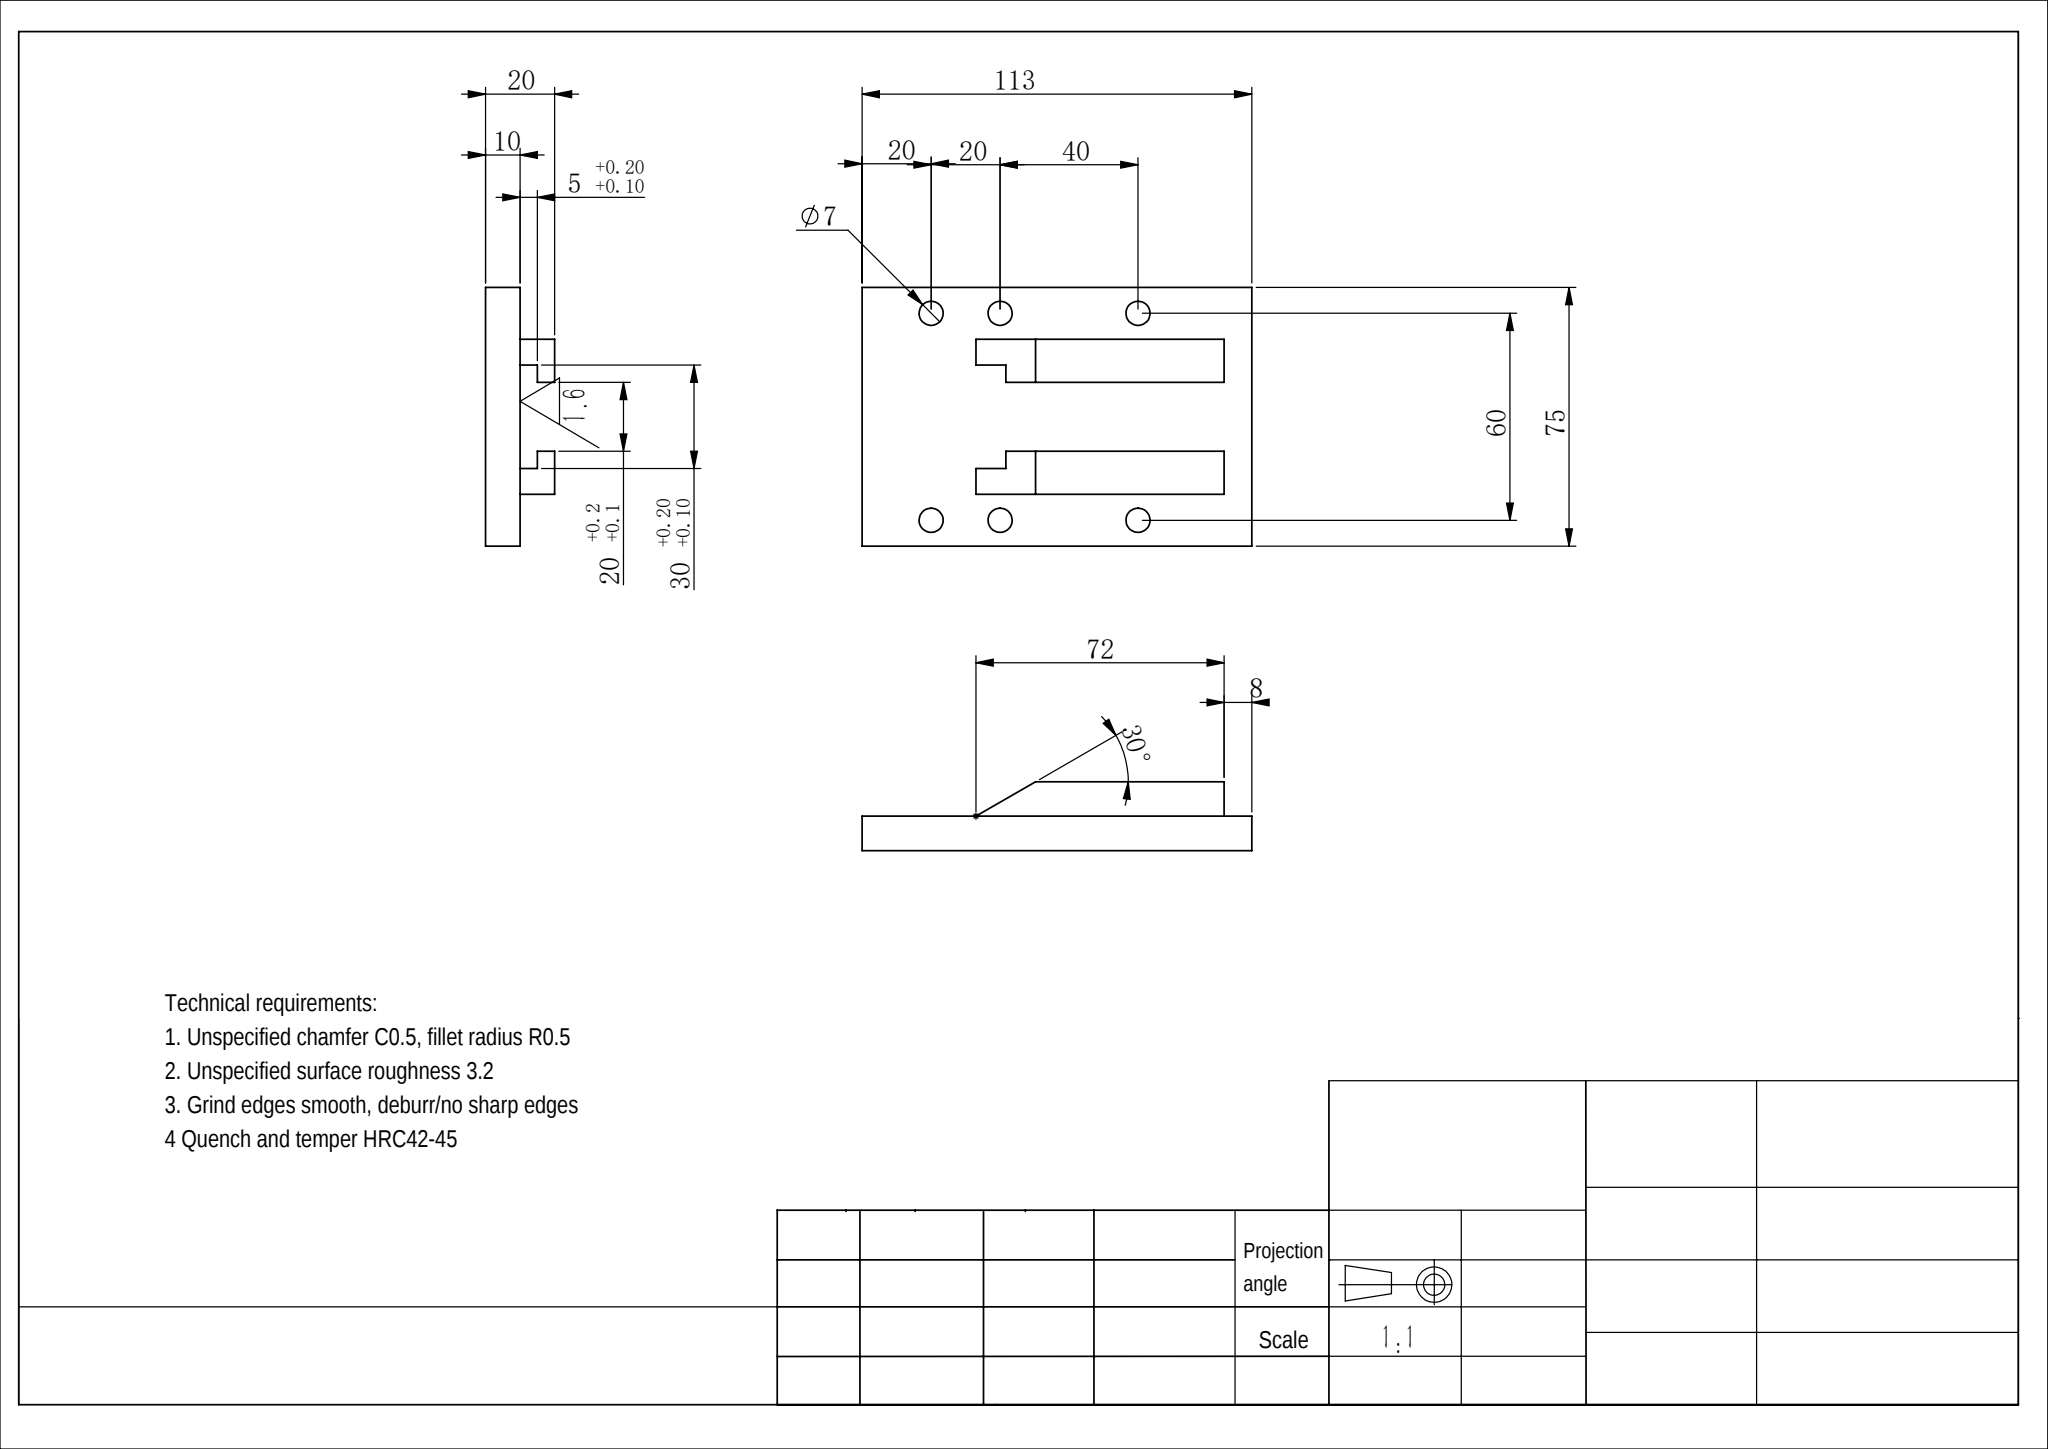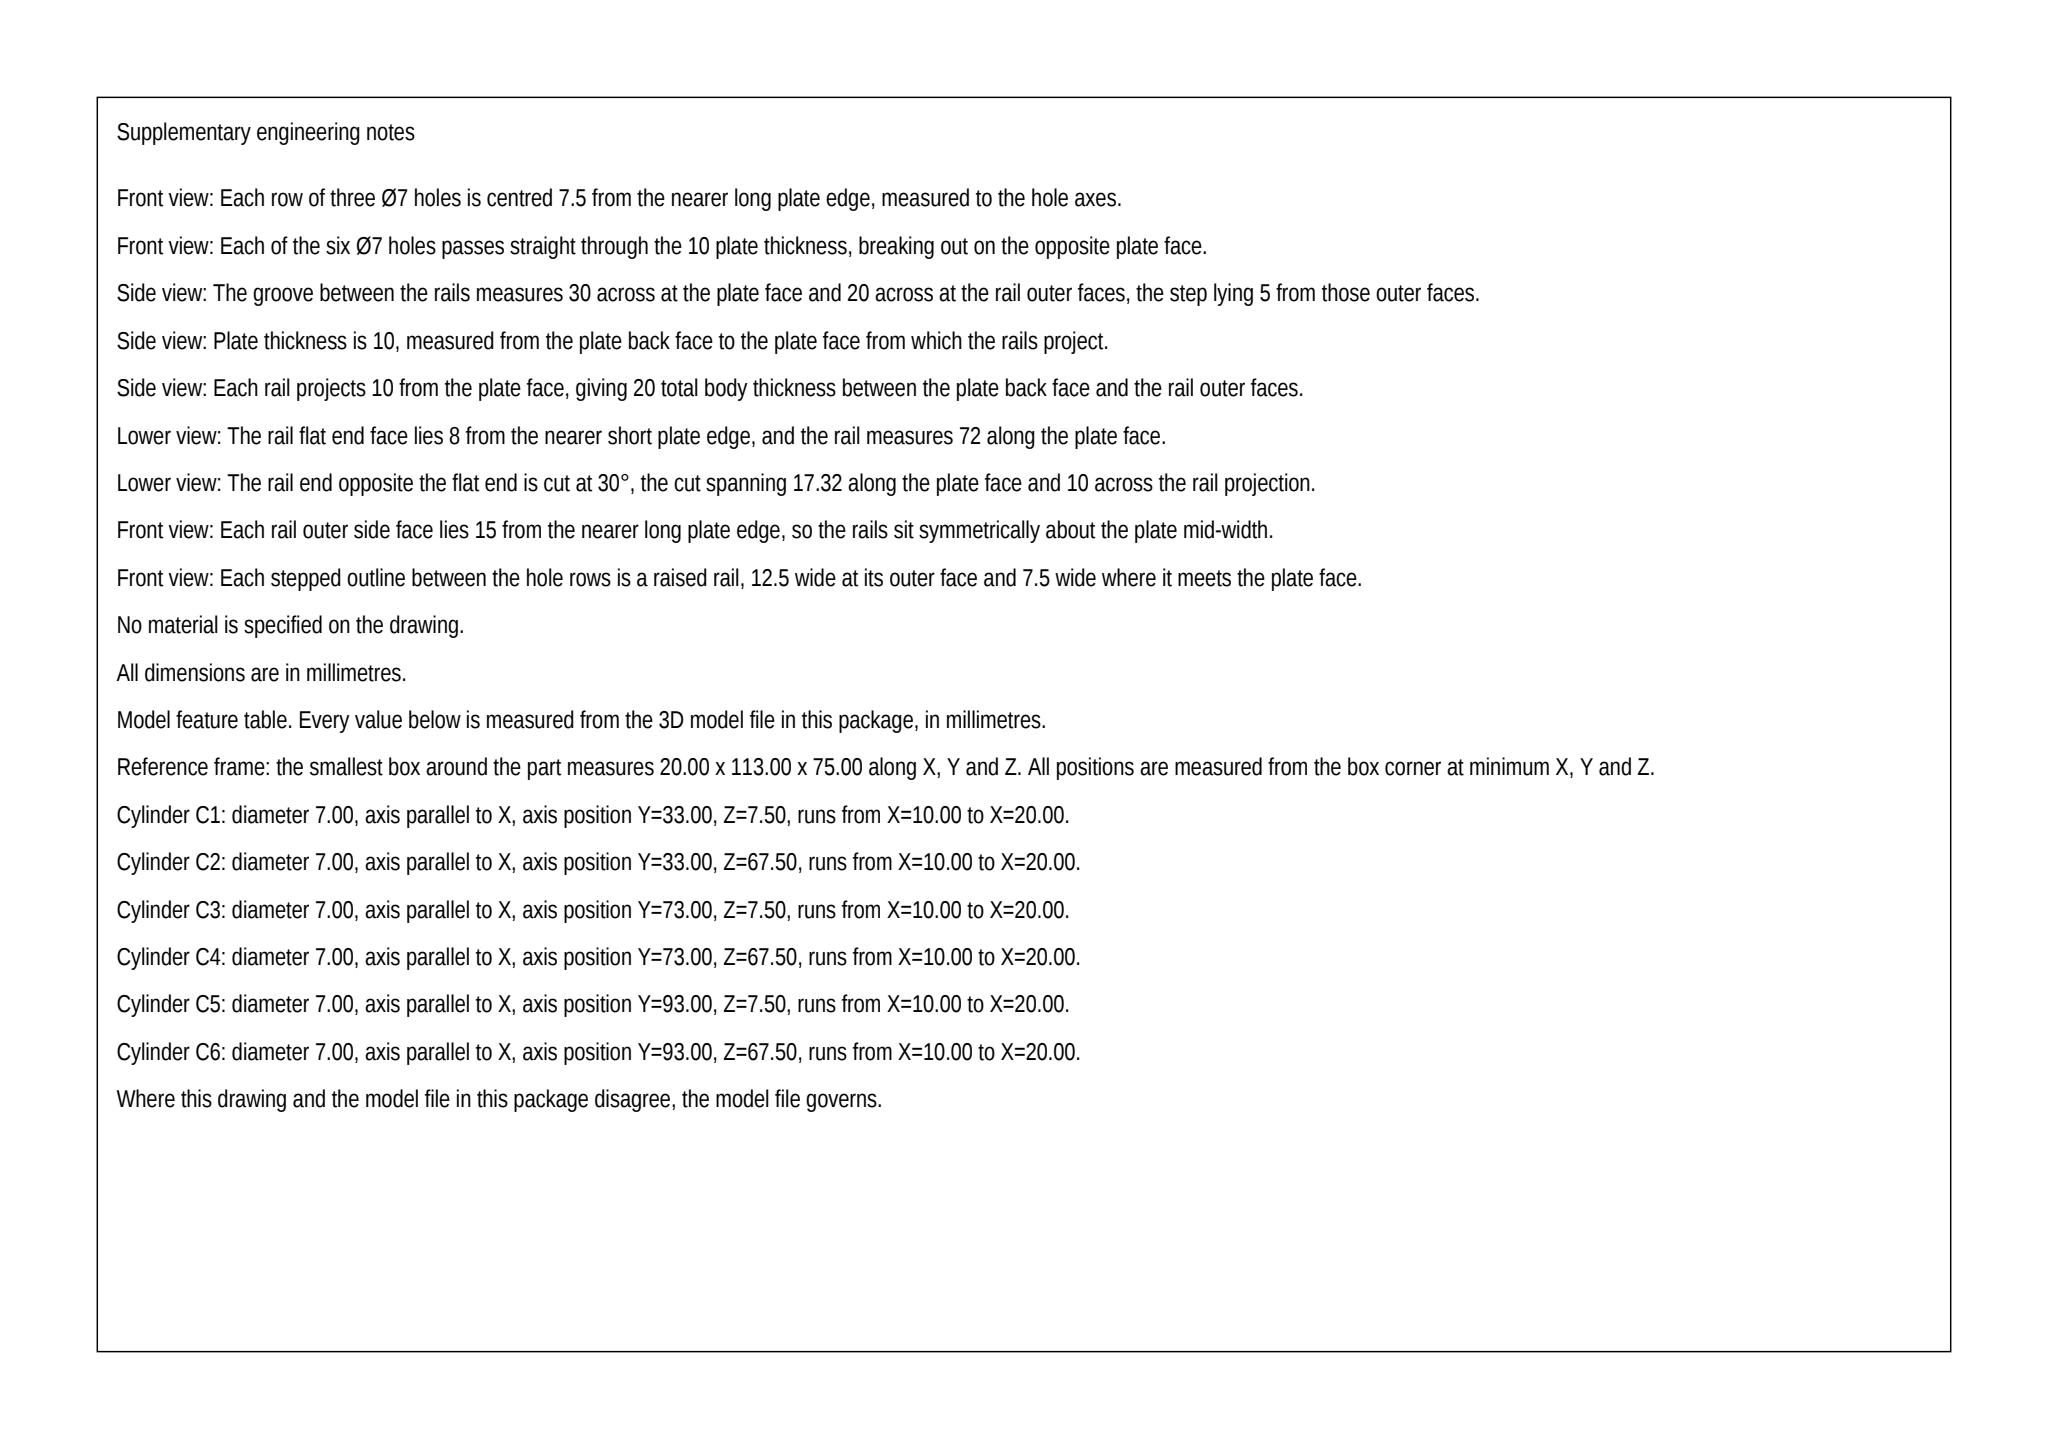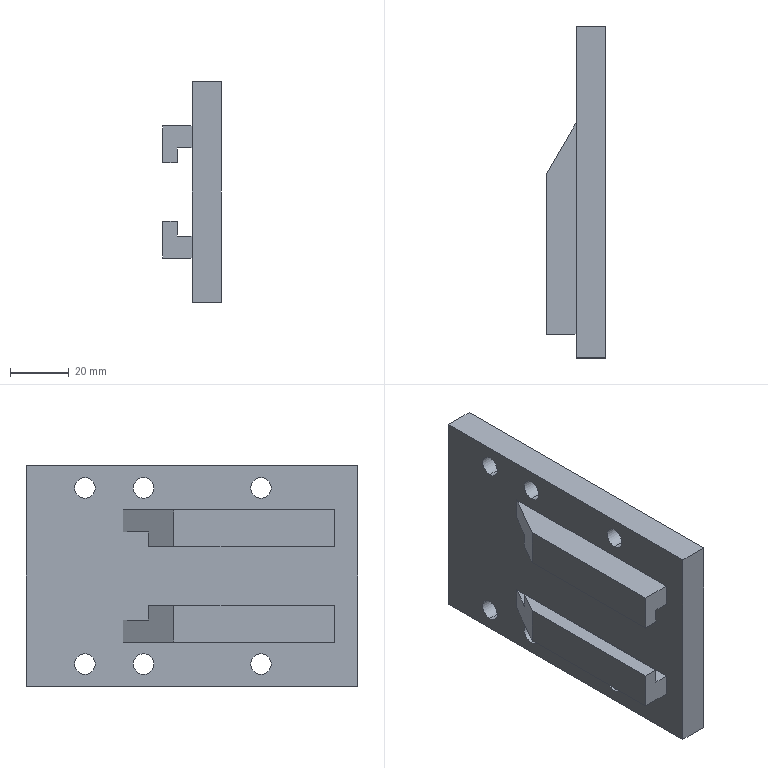Part | SolidWorks | mm | 1 solid | 32 faces | box 20 x 113 x 75 mm | volume 94892 mm3 | plane 20 | cylinder 12 | commonest cylinder face diameters 7 x12
Drawing notes:
2X SLOT SYM ABOUT CL OF 75; SLOT CL 12.5 EA SIDE OF CL | from the solid: z planes 22.5/27.5 & 47.5/52.5 -> slot CLs 25 & 50, sym about 37.5 = 75/2
SLOT WIDTH 5 (Z) 2X; 22.5 FROM BOTTOM EDGE TO 1ST SLOT | from the solid: z planes 22.5,27.5,47.5,52.5 give 5 wide slots; first face 22.5 from z=0
SLOT STEP DEPTH: 5 DEEP STEP IN 10 DEEP SLOT (X 0-5-10) | from the solid: x planes at 0, 5, 10, 20 (bbox x=20)
BOTH SLOTS: DP 5 STEP 8 LG FROM RH EDGE, BAL DP 10 | from the solid: y-planes at 0/8/113 (y=8 x2 = slot step faces); x-planes at 5 and 10 give the 5 and 10 depths; 113 overall in Y
6X Ø7 THRU 10 THK FLANGE; 2 ROWS, HOLE CL 7.5 FROM BOTTOM EDGE AND 7.5 FROM TOP EDGE (67.5 FROM BOTTOM) OF 75 | from the solid: cylinders dia 7.0, axis x, length 10.0 at z=7.5 and z=67.5 (6 holes total)
HOLE COLUMNS AT 33, 73 AND 93 FROM LEFT (Y=0) EDGE OF 113 | from the solid: cylinders dia 7.0 positions y=33.0, 73.0, 93.0
PROFILE STEP FACES AT 15 FROM BOTTOM EDGE AND 15 FROM TOP EDGE (Z=15 AND Z=60) OF 75 | from the solid: axis_planes normal z at offsets 15.0 and 60.0
2X SLOT 5 WIDE (Z 22.5-27.5 AND 47.5-52.5), 10 DP, OPEN-ENDED: RUNS FULL 113 LG FROM Y=0 EDGE THRU Y=113 EDGE; 5 DP STEP FACE AT Y=8 FROM Y=0 EDGE | from the solid: axis_planes y-normal exist only at y=0, y=8 (count 2 = one step face per slot) and y=113 - no slot end faces; z planes 22.5/27.5 and 47.5/52.5 give the two 5 wide slots
8 THK UPRIGHT LEG FLUSH WITH Y=0 EDGE OF 113; INNER FACE OF LEG AT Y=8 FROM Y=0 DATUM EDGE | from the solid: axis_planes y-normal at y=0.0 and y=8.0 with bbox_xyz y=113.0
build123d program:
from build123d import *

# Parameters (mm, degrees)
SKETCH1_W           = 75
SKETCH1_H           = 113
BOSS_EXTRUDE1_DEPTH = 10
SKETCH5_W           = 45
SKETCH5_H           = 80
BOSS_EXTRUDE4_DEPTH = 10
CUT_EXTRUDE2_DEPTH  = 84.02
CUT_EXTRUDE3_DEPTH  = 120.479
SKETCH8_W           = 45
SKETCH8_H           = 8
CUT_EXTRUDE4_DEPTH  = 30
SKETCH9_R           = 3.5
CUT_EXTRUDE5_DEPTH  = 30


with BuildPart() as part:
    # Sketch1 → Boss-Extrude1 (new body)
    with BuildSketch(Plane(origin=(0, 0, 0), x_dir=(0, 0, -1), z_dir=(1, 0, 0))):
        Rectangle(SKETCH1_W, SKETCH1_H)
    extrude(amount=BOSS_EXTRUDE1_DEPTH)

    # Sketch5 → Boss-Extrude4 (add)
    with BuildSketch(Plane.ZY):
        with Locations((0, -16.5)):
            Rectangle(SKETCH5_W, SKETCH5_H)
    extrude(amount=BOSS_EXTRUDE4_DEPTH)

    # Sketch6 → Cut-Extrude2 (cut, through all)
    with BuildSketch(Plane.XY.offset(22.5)):
        Polygon((0, 23.5), (-10, 6.179), (-10, 23.5), align=None)
    extrude(amount=-CUT_EXTRUDE2_DEPTH, mode=Mode.SUBTRACT)

    # Sketch7 → Cut-Extrude3 (cut, through all)
    with BuildSketch(Plane.XZ.offset(56.5)):
        Polygon((-10, 10), (-5, 10), (-5, 15), (0, 15), (0, -15), (-5, -15), (-5, -10), (-10, -10), align=None)
    extrude(amount=-CUT_EXTRUDE3_DEPTH, mode=Mode.SUBTRACT)

    # Sketch8 → Cut-Extrude4 (cut)
    with BuildSketch(Plane.ZY):
        with Locations((0, -52.5)):
            Rectangle(SKETCH8_W, SKETCH8_H)
    extrude(amount=CUT_EXTRUDE4_DEPTH, mode=Mode.SUBTRACT)

    # Sketch9 → Cut-Extrude5 (cut)
    with BuildSketch(Plane(origin=(10, 0, 0), x_dir=(0, 0, -1), z_dir=(1, 0, 0))):
        with Locations((30, 36.5)):
            Circle(SKETCH9_R)
        with Locations((30, 16.5)):
            Circle(SKETCH9_R)
        with Locations((30, -23.5)):
            Circle(SKETCH9_R)
        with Locations((-30, 36.5)):
            Circle(SKETCH9_R)
        with Locations((-30, 16.5)):
            Circle(SKETCH9_R)
        with Locations((-30, -23.5)):
            Circle(SKETCH9_R)
    extrude(amount=-CUT_EXTRUDE5_DEPTH, mode=Mode.SUBTRACT)


solid = part.part